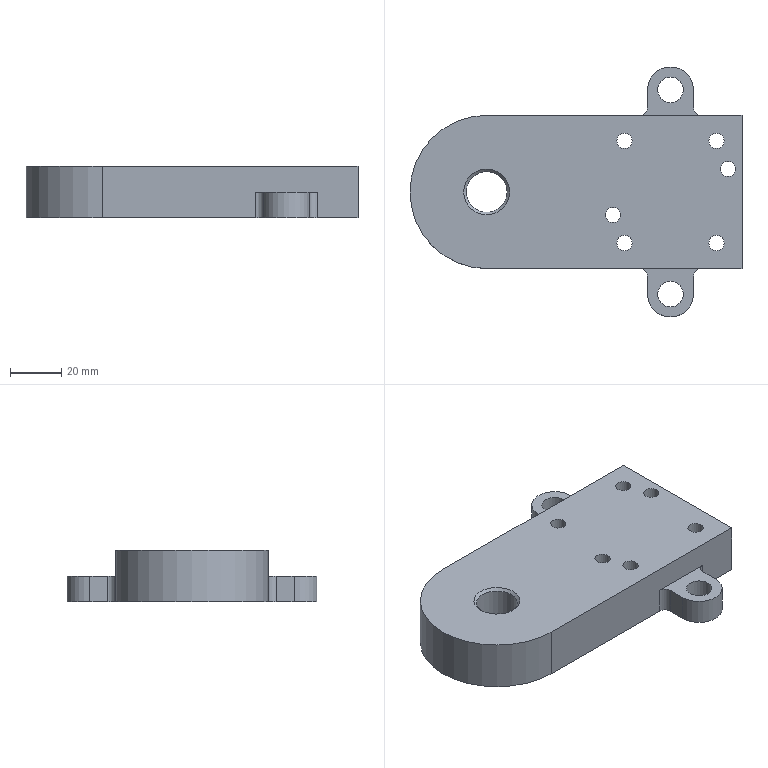Component | NX | BASE | 1 solid | 28 faces | volume 145485 mm3 | cylinder 16 | plane 11 | cone 1 | commonest cylinder face diameters 6 x10 18 x2 10 x2 60 x1 16 x1